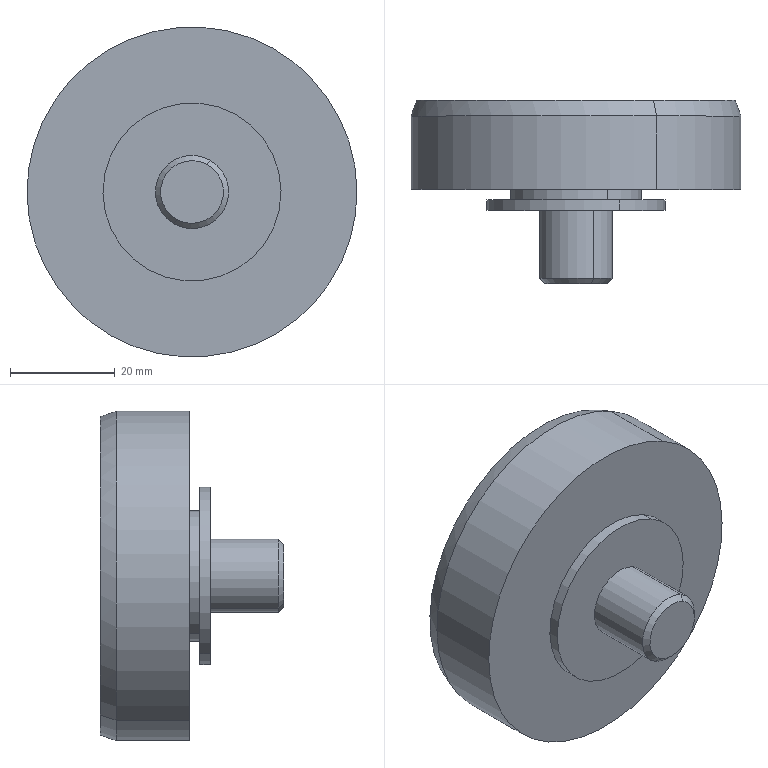Component | SolidWorks | LocatingPinAxis-1 | 1 solid | 17 faces | box 63 x 35 x 63 mm | volume 57605 mm3 | cylinder 8 | plane 5 | cone 4 | commonest cylinder face diameters 14 x2 34 x2 25 x2 63 x2
build123d program:
from build123d import *

# Parameters (mm, degrees)
CHAMFER1_SIZE  = 3
CHAMFER1_SIZE2 = 1.092
CHAMFER2_SIZE  = 1


with BuildPart() as part:
    # Sketch1 → Revolve1 (revolve)
    with BuildSketch(Plane.XY, mode=Mode.PRIVATE) as revolve1_sk:
        Polygon((0, 0), (31.5, 0), (31.5, -17), (12.5, -17), (12.5, -19), (17, -19), (17, -21), (7, -21), (7, -35), (0, -35), align=None)
    revolve(revolve1_sk.sketch.rotate(Axis((0, -35, 0), (0, 1, 0)), 90), axis=Axis((0, -35, 0), (0, 1, 0)))

    # Chamfer1
    chamfer1_edges = [part.edges().sort_by_distance(p)[0] for p in [
        (0, 0, 31.5),
    ]]
    chamfer1_side = [part.faces().sort_by_distance(p)[0] for p in [
        (0, -8.5, 31.5),
    ]]
    chamfer(chamfer1_edges, length=CHAMFER1_SIZE, length2=CHAMFER1_SIZE2, reference=chamfer1_side[0])

    # Chamfer2
    chamfer2_edges = [part.edges().sort_by_distance(p)[0] for p in [
        (0, -35, 7),
    ]]
    chamfer(chamfer2_edges, length=CHAMFER2_SIZE)


solid = part.part

# Placed as in the assembly
solid = solid.moved(Location((0, 226.806, 0), (0, 0, 0)))
STEP:
#1=CARTESIAN_POINT('',(-0.1151,7.551,-0.2063));
#2=VERTEX_POINT('',#1);
#3=CARTESIAN_POINT('',(0.1151,7.551,0.2063));
#4=VERTEX_POINT('',#3);
#5=CARTESIAN_POINT('',(-0.,7.551,0.));
#6=DIRECTION('',(0.,-1.,0.));
#7=DIRECTION('',(-0.4873,0.,-0.8733));
#8=AXIS2_PLACEMENT_3D('',#5,#6,#7);
#9=CIRCLE('',#8,0.2362);
#10=EDGE_CURVE('',#2,#4,#9,.T.);
#11=ORIENTED_EDGE('',*,*,#10,.F.);
#12=CARTESIAN_POINT('',(-0.1343,7.591,-0.2407));
#13=VERTEX_POINT('',#12);
#14=CARTESIAN_POINT('',(-0.1151,7.551,-0.2063));
#15=DIRECTION('',(-0.3445,0.7071,-0.6175));
#16=VECTOR('',#15,39.37);
#17=LINE('',#14,#16);
#18=EDGE_CURVE('',#2,#13,#17,.T.);
#19=ORIENTED_EDGE('',*,*,#18,.T.);
#20=CARTESIAN_POINT('',(0.1343,7.591,0.2407));
#21=VERTEX_POINT('',#20);
#22=CARTESIAN_POINT('',(-0.,7.591,0.));
#23=DIRECTION('',(0.,1.,0.));
#24=DIRECTION('',(-0.4873,0.,-0.8733));
#25=AXIS2_PLACEMENT_3D('',#22,#23,#24);
#26=CIRCLE('',#25,0.2756);
#27=EDGE_CURVE('',#21,#13,#26,.T.);
#28=ORIENTED_EDGE('',*,*,#27,.F.);
#29=CARTESIAN_POINT('',(0.1151,7.551,0.2063));
#30=DIRECTION('',(0.3445,0.7071,0.6175));
#31=VECTOR('',#30,39.37);
#32=LINE('',#29,#31);
#33=EDGE_CURVE('',#4,#21,#32,.T.);
#34=ORIENTED_EDGE('',*,*,#33,.F.);
#35=EDGE_LOOP('',(#11,#19,#28,#34));
#36=FACE_OUTER_BOUND('',#35,.T.);
#37=CARTESIAN_POINT('',(-0.,7.551,0.));
#38=DIRECTION('',(0.,1.,0.));
#39=DIRECTION('',(0.4873,0.,0.8733));
#40=AXIS2_PLACEMENT_3D('',#37,#38,#39);
#41=CONICAL_SURFACE('',#40,0.2362,0.7854);
#42=ADVANCED_FACE('',(#36),#41,.T.);
#43=CARTESIAN_POINT('',(0.5833,8.929,1.045));
#44=VERTEX_POINT('',#43);
#45=CARTESIAN_POINT('',(-0.5833,8.929,-1.045));
#46=VERTEX_POINT('',#45);
#47=CARTESIAN_POINT('',(-0.,8.929,0.));
#48=DIRECTION('',(0.,1.,0.));
#49=DIRECTION('',(0.4873,0.,0.8733));
#50=AXIS2_PLACEMENT_3D('',#47,#48,#49);
#51=CIRCLE('',#50,1.197);
#52=EDGE_CURVE('',#44,#46,#51,.T.);
#53=ORIENTED_EDGE('',*,*,#52,.F.);
#54=CARTESIAN_POINT('',(0.6043,8.811,1.083));
#55=VERTEX_POINT('',#54);
#56=CARTESIAN_POINT('',(0.6043,8.811,1.083));
#57=DIRECTION('',(0.1667,-0.9397,0.2987));
#58=VECTOR('',#57,39.37);
#59=LINE('',#56,#58);
#60=EDGE_CURVE('',#44,#55,#59,.T.);
#61=ORIENTED_EDGE('',*,*,#60,.T.);
#62=CARTESIAN_POINT('',(-0.6043,8.811,-1.083));
#63=VERTEX_POINT('',#62);
#64=CARTESIAN_POINT('',(-0.,8.811,0.));
#65=DIRECTION('',(0.,-1.,0.));
#66=DIRECTION('',(0.4873,0.,0.8733));
#67=AXIS2_PLACEMENT_3D('',#64,#65,#66);
#68=CIRCLE('',#67,1.24);
#69=EDGE_CURVE('',#63,#55,#68,.T.);
#70=ORIENTED_EDGE('',*,*,#69,.F.);
#71=CARTESIAN_POINT('',(-0.6043,8.811,-1.083));
#72=DIRECTION('',(-0.1667,-0.9397,-0.2987));
#73=VECTOR('',#72,39.37);
#74=LINE('',#71,#73);
#75=EDGE_CURVE('',#46,#63,#74,.T.);
#76=ORIENTED_EDGE('',*,*,#75,.F.);
#77=EDGE_LOOP('',(#53,#61,#70,#76));
#78=FACE_OUTER_BOUND('',#77,.T.);
#79=CARTESIAN_POINT('',(-0.,8.811,0.));
#80=DIRECTION('',(0.,-1.,0.));
#81=DIRECTION('',(-0.4873,0.,-0.8733));
#82=AXIS2_PLACEMENT_3D('',#79,#80,#81);
#83=CONICAL_SURFACE('',#82,1.24,0.3491);
#84=ADVANCED_FACE('',(#78),#83,.T.);
#85=CARTESIAN_POINT('',(-0.1343,8.103,-0.2407));
#86=VERTEX_POINT('',#85);
#87=CARTESIAN_POINT('',(0.1343,8.103,0.2407));
#88=VERTEX_POINT('',#87);
#89=CARTESIAN_POINT('',(-0.,8.103,0.));
#90=DIRECTION('',(0.,-1.,0.));
#91=DIRECTION('',(-0.4873,0.,-0.8733));
#92=AXIS2_PLACEMENT_3D('',#89,#90,#91);
#93=CIRCLE('',#92,0.2756);
#94=EDGE_CURVE('',#86,#88,#93,.T.);
#95=ORIENTED_EDGE('',*,*,#94,.T.);
#96=CARTESIAN_POINT('',(0.1343,7.551,0.2407));
#97=DIRECTION('',(0.,-1.,0.));
#98=VECTOR('',#97,39.37);
#99=LINE('',#96,#98);
#100=EDGE_CURVE('',#88,#21,#99,.T.);
#101=ORIENTED_EDGE('',*,*,#100,.T.);
#102=ORIENTED_EDGE('',*,*,#27,.T.);
#103=CARTESIAN_POINT('',(-0.1343,7.551,-0.2407));
#104=DIRECTION('',(0.,-1.,0.));
#105=VECTOR('',#104,39.37);
#106=LINE('',#103,#105);
#107=EDGE_CURVE('',#86,#13,#106,.T.);
#108=ORIENTED_EDGE('',*,*,#107,.F.);
#109=EDGE_LOOP('',(#95,#101,#102,#108));
#110=FACE_OUTER_BOUND('',#109,.T.);
#111=CARTESIAN_POINT('',(-0.,7.551,0.));
#112=DIRECTION('',(0.,-1.,0.));
#113=DIRECTION('',(-0.4873,0.,-0.8733));
#114=AXIS2_PLACEMENT_3D('',#111,#112,#113);
#115=CYLINDRICAL_SURFACE('',#114,0.2756);
#116=ADVANCED_FACE('',(#110),#115,.T.);
#117=CARTESIAN_POINT('',(-0.3261,8.181,-0.5845));
#118=VERTEX_POINT('',#117);
#119=CARTESIAN_POINT('',(0.3261,8.181,0.5845));
#120=VERTEX_POINT('',#119);
#121=CARTESIAN_POINT('',(-0.,8.181,0.));
#122=DIRECTION('',(0.,-1.,0.));
#123=DIRECTION('',(-0.4873,0.,-0.8733));
#124=AXIS2_PLACEMENT_3D('',#121,#122,#123);
#125=CIRCLE('',#124,0.6693);
#126=EDGE_CURVE('',#118,#120,#125,.T.);
#127=ORIENTED_EDGE('',*,*,#126,.T.);
#128=CARTESIAN_POINT('',(0.3261,8.103,0.5845));
#129=VERTEX_POINT('',#128);
#130=CARTESIAN_POINT('',(0.3261,7.551,0.5845));
#131=DIRECTION('',(0.,-1.,0.));
#132=VECTOR('',#131,39.37);
#133=LINE('',#130,#132);
#134=EDGE_CURVE('',#120,#129,#133,.T.);
#135=ORIENTED_EDGE('',*,*,#134,.T.);
#136=CARTESIAN_POINT('',(-0.3261,8.103,-0.5845));
#137=VERTEX_POINT('',#136);
#138=CARTESIAN_POINT('',(-0.,8.103,0.));
#139=DIRECTION('',(0.,-1.,0.));
#140=DIRECTION('',(-0.4873,0.,-0.8733));
#141=AXIS2_PLACEMENT_3D('',#138,#139,#140);
#142=CIRCLE('',#141,0.6693);
#143=EDGE_CURVE('',#137,#129,#142,.T.);
#144=ORIENTED_EDGE('',*,*,#143,.F.);
#145=CARTESIAN_POINT('',(-0.3261,7.551,-0.5845));
#146=DIRECTION('',(0.,-1.,0.));
#147=VECTOR('',#146,39.37);
#148=LINE('',#145,#147);
#149=EDGE_CURVE('',#118,#137,#148,.T.);
#150=ORIENTED_EDGE('',*,*,#149,.F.);
#151=EDGE_LOOP('',(#127,#135,#144,#150));
#152=FACE_OUTER_BOUND('',#151,.T.);
#153=CARTESIAN_POINT('',(-0.,7.551,0.));
#154=DIRECTION('',(0.,-1.,0.));
#155=DIRECTION('',(-0.4873,0.,-0.8733));
#156=AXIS2_PLACEMENT_3D('',#153,#154,#155);
#157=CYLINDRICAL_SURFACE('',#156,0.6693);
#158=ADVANCED_FACE('',(#152),#157,.T.);
#159=CARTESIAN_POINT('',(-0.2398,8.26,-0.4298));
#160=VERTEX_POINT('',#159);
#161=CARTESIAN_POINT('',(0.2398,8.26,0.4298));
#162=VERTEX_POINT('',#161);
#163=CARTESIAN_POINT('',(-0.,8.26,0.));
#164=DIRECTION('',(0.,-1.,0.));
#165=DIRECTION('',(-0.4873,0.,-0.8733));
#166=AXIS2_PLACEMENT_3D('',#163,#164,#165);
#167=CIRCLE('',#166,0.4921);
#168=EDGE_CURVE('',#160,#162,#167,.T.);
#169=ORIENTED_EDGE('',*,*,#168,.T.);
#170=CARTESIAN_POINT('',(0.2398,8.181,0.4298));
#171=VERTEX_POINT('',#170);
#172=CARTESIAN_POINT('',(0.2398,7.551,0.4298));
#173=DIRECTION('',(0.,-1.,0.));
#174=VECTOR('',#173,39.37);
#175=LINE('',#172,#174);
#176=EDGE_CURVE('',#162,#171,#175,.T.);
#177=ORIENTED_EDGE('',*,*,#176,.T.);
#178=CARTESIAN_POINT('',(-0.2398,8.181,-0.4298));
#179=VERTEX_POINT('',#178);
#180=CARTESIAN_POINT('',(-0.,8.181,0.));
#181=DIRECTION('',(0.,-1.,0.));
#182=DIRECTION('',(-0.4873,0.,-0.8733));
#183=AXIS2_PLACEMENT_3D('',#180,#181,#182);
#184=CIRCLE('',#183,0.4921);
#185=EDGE_CURVE('',#179,#171,#184,.T.);
#186=ORIENTED_EDGE('',*,*,#185,.F.);
#187=CARTESIAN_POINT('',(-0.2398,7.551,-0.4298));
#188=DIRECTION('',(0.,-1.,0.));
#189=VECTOR('',#188,39.37);
#190=LINE('',#187,#189);
#191=EDGE_CURVE('',#160,#179,#190,.T.);
#192=ORIENTED_EDGE('',*,*,#191,.F.);
#193=EDGE_LOOP('',(#169,#177,#186,#192));
#194=FACE_OUTER_BOUND('',#193,.T.);
#195=CARTESIAN_POINT('',(-0.,7.551,0.));
#196=DIRECTION('',(0.,-1.,0.));
#197=DIRECTION('',(-0.4873,0.,-0.8733));
#198=AXIS2_PLACEMENT_3D('',#195,#196,#197);
#199=CYLINDRICAL_SURFACE('',#198,0.4921);
#200=ADVANCED_FACE('',(#194),#199,.T.);
#201=ORIENTED_EDGE('',*,*,#69,.T.);
#202=CARTESIAN_POINT('',(0.6043,8.26,1.083));
#203=VERTEX_POINT('',#202);
#204=CARTESIAN_POINT('',(0.6043,7.551,1.083));
#205=DIRECTION('',(0.,-1.,0.));
#206=VECTOR('',#205,39.37);
#207=LINE('',#204,#206);
#208=EDGE_CURVE('',#55,#203,#207,.T.);
#209=ORIENTED_EDGE('',*,*,#208,.T.);
#210=CARTESIAN_POINT('',(-0.6043,8.26,-1.083));
#211=VERTEX_POINT('',#210);
#212=CARTESIAN_POINT('',(-0.,8.26,0.));
#213=DIRECTION('',(0.,-1.,0.));
#214=DIRECTION('',(-0.4873,0.,-0.8733));
#215=AXIS2_PLACEMENT_3D('',#212,#213,#214);
#216=CIRCLE('',#215,1.24);
#217=EDGE_CURVE('',#211,#203,#216,.T.);
#218=ORIENTED_EDGE('',*,*,#217,.F.);
#219=CARTESIAN_POINT('',(-0.6043,7.551,-1.083));
#220=DIRECTION('',(0.,-1.,0.));
#221=VECTOR('',#220,39.37);
#222=LINE('',#219,#221);
#223=EDGE_CURVE('',#63,#211,#222,.T.);
#224=ORIENTED_EDGE('',*,*,#223,.F.);
#225=EDGE_LOOP('',(#201,#209,#218,#224));
#226=FACE_OUTER_BOUND('',#225,.T.);
#227=CARTESIAN_POINT('',(-0.,7.551,0.));
#228=DIRECTION('',(0.,-1.,0.));
#229=DIRECTION('',(-0.4873,0.,-0.8733));
#230=AXIS2_PLACEMENT_3D('',#227,#228,#229);
#231=CYLINDRICAL_SURFACE('',#230,1.24);
#232=ADVANCED_FACE('',(#226),#231,.T.);
#233=CARTESIAN_POINT('',(-0.,8.929,0.));
#234=DIRECTION('',(0.,1.,0.));
#235=DIRECTION('',(0.4873,0.,0.8733));
#236=AXIS2_PLACEMENT_3D('',#233,#234,#235);
#237=CIRCLE('',#236,1.197);
#238=EDGE_CURVE('',#46,#44,#237,.T.);
#239=ORIENTED_EDGE('',*,*,#238,.T.);
#240=ORIENTED_EDGE('',*,*,#52,.T.);
#241=EDGE_LOOP('',(#239,#240));
#242=FACE_OUTER_BOUND('',#241,.T.);
#243=CARTESIAN_POINT('',(-0.,8.929,0.));
#244=DIRECTION('',(0.,1.,0.));
#245=DIRECTION('',(0.4873,0.,0.8733));
#246=AXIS2_PLACEMENT_3D('',#243,#244,#245);
#247=PLANE('',#246);
#248=ADVANCED_FACE('',(#242),#247,.T.);
#249=ORIENTED_EDGE('',*,*,#208,.F.);
#250=CARTESIAN_POINT('',(-0.,8.811,0.));
#251=DIRECTION('',(0.,-1.,0.));
#252=DIRECTION('',(0.4873,0.,0.8733));
#253=AXIS2_PLACEMENT_3D('',#250,#251,#252);
#254=CIRCLE('',#253,1.24);
#255=EDGE_CURVE('',#55,#63,#254,.T.);
#256=ORIENTED_EDGE('',*,*,#255,.T.);
#257=ORIENTED_EDGE('',*,*,#223,.T.);
#258=CARTESIAN_POINT('',(-0.,8.26,0.));
#259=DIRECTION('',(0.,-1.,0.));
#260=DIRECTION('',(-0.4873,0.,-0.8733));
#261=AXIS2_PLACEMENT_3D('',#258,#259,#260);
#262=CIRCLE('',#261,1.24);
#263=EDGE_CURVE('',#203,#211,#262,.T.);
#264=ORIENTED_EDGE('',*,*,#263,.F.);
#265=EDGE_LOOP('',(#249,#256,#257,#264));
#266=FACE_OUTER_BOUND('',#265,.T.);
#267=CARTESIAN_POINT('',(-0.,7.551,0.));
#268=DIRECTION('',(0.,-1.,0.));
#269=DIRECTION('',(-0.4873,0.,-0.8733));
#270=AXIS2_PLACEMENT_3D('',#267,#268,#269);
#271=CYLINDRICAL_SURFACE('',#270,1.24);
#272=ADVANCED_FACE('',(#266),#271,.T.);
#273=ORIENTED_EDGE('',*,*,#217,.T.);
#274=ORIENTED_EDGE('',*,*,#263,.T.);
#275=EDGE_LOOP('',(#273,#274));
#276=FACE_OUTER_BOUND('',#275,.T.);
#277=ORIENTED_EDGE('',*,*,#168,.F.);
#278=CARTESIAN_POINT('',(-0.,8.26,0.));
#279=DIRECTION('',(0.,-1.,0.));
#280=DIRECTION('',(-0.4873,0.,-0.8733));
#281=AXIS2_PLACEMENT_3D('',#278,#279,#280);
#282=CIRCLE('',#281,0.4921);
#283=EDGE_CURVE('',#162,#160,#282,.T.);
#284=ORIENTED_EDGE('',*,*,#283,.F.);
#285=EDGE_LOOP('',(#277,#284));
#286=FACE_BOUND('',#285,.T.);
#287=CARTESIAN_POINT('',(0.4298,8.26,-0.2398));
#288=DIRECTION('',(0.,-1.,0.));
#289=DIRECTION('',(-0.4873,0.,-0.8733));
#290=AXIS2_PLACEMENT_3D('',#287,#288,#289);
#291=PLANE('',#290);
#292=ADVANCED_FACE('',(#276,#286),#291,.T.);
#293=ORIENTED_EDGE('',*,*,#176,.F.);
#294=ORIENTED_EDGE('',*,*,#283,.T.);
#295=ORIENTED_EDGE('',*,*,#191,.T.);
#296=CARTESIAN_POINT('',(-0.,8.181,0.));
#297=DIRECTION('',(0.,-1.,0.));
#298=DIRECTION('',(-0.4873,0.,-0.8733));
#299=AXIS2_PLACEMENT_3D('',#296,#297,#298);
#300=CIRCLE('',#299,0.4921);
#301=EDGE_CURVE('',#171,#179,#300,.T.);
#302=ORIENTED_EDGE('',*,*,#301,.F.);
#303=EDGE_LOOP('',(#293,#294,#295,#302));
#304=FACE_OUTER_BOUND('',#303,.T.);
#305=CARTESIAN_POINT('',(-0.,7.551,0.));
#306=DIRECTION('',(0.,-1.,0.));
#307=DIRECTION('',(-0.4873,0.,-0.8733));
#308=AXIS2_PLACEMENT_3D('',#305,#306,#307);
#309=CYLINDRICAL_SURFACE('',#308,0.4921);
#310=ADVANCED_FACE('',(#304),#309,.T.);
#311=ORIENTED_EDGE('',*,*,#185,.T.);
#312=ORIENTED_EDGE('',*,*,#301,.T.);
#313=EDGE_LOOP('',(#311,#312));
#314=FACE_BOUND('',#313,.T.);
#315=ORIENTED_EDGE('',*,*,#126,.F.);
#316=CARTESIAN_POINT('',(-0.,8.181,0.));
#317=DIRECTION('',(0.,-1.,0.));
#318=DIRECTION('',(-0.4873,0.,-0.8733));
#319=AXIS2_PLACEMENT_3D('',#316,#317,#318);
#320=CIRCLE('',#319,0.6693);
#321=EDGE_CURVE('',#120,#118,#320,.T.);
#322=ORIENTED_EDGE('',*,*,#321,.F.);
#323=EDGE_LOOP('',(#315,#322));
#324=FACE_OUTER_BOUND('',#323,.T.);
#325=CARTESIAN_POINT('',(0.4298,8.181,-0.2398));
#326=DIRECTION('',(0.,1.,0.));
#327=DIRECTION('',(0.4873,0.,0.8733));
#328=AXIS2_PLACEMENT_3D('',#325,#326,#327);
#329=PLANE('',#328);
#330=ADVANCED_FACE('',(#314,#324),#329,.T.);
#331=ORIENTED_EDGE('',*,*,#134,.F.);
#332=ORIENTED_EDGE('',*,*,#321,.T.);
#333=ORIENTED_EDGE('',*,*,#149,.T.);
#334=CARTESIAN_POINT('',(-0.,8.103,0.));
#335=DIRECTION('',(0.,-1.,0.));
#336=DIRECTION('',(-0.4873,0.,-0.8733));
#337=AXIS2_PLACEMENT_3D('',#334,#335,#336);
#338=CIRCLE('',#337,0.6693);
#339=EDGE_CURVE('',#129,#137,#338,.T.);
#340=ORIENTED_EDGE('',*,*,#339,.F.);
#341=EDGE_LOOP('',(#331,#332,#333,#340));
#342=FACE_OUTER_BOUND('',#341,.T.);
#343=CARTESIAN_POINT('',(-0.,7.551,0.));
#344=DIRECTION('',(0.,-1.,0.));
#345=DIRECTION('',(-0.4873,0.,-0.8733));
#346=AXIS2_PLACEMENT_3D('',#343,#344,#345);
#347=CYLINDRICAL_SURFACE('',#346,0.6693);
#348=ADVANCED_FACE('',(#342),#347,.T.);
#349=ORIENTED_EDGE('',*,*,#143,.T.);
#350=ORIENTED_EDGE('',*,*,#339,.T.);
#351=EDGE_LOOP('',(#349,#350));
#352=FACE_OUTER_BOUND('',#351,.T.);
#353=ORIENTED_EDGE('',*,*,#94,.F.);
#354=CARTESIAN_POINT('',(-0.,8.103,0.));
#355=DIRECTION('',(0.,-1.,0.));
#356=DIRECTION('',(-0.4873,0.,-0.8733));
#357=AXIS2_PLACEMENT_3D('',#354,#355,#356);
#358=CIRCLE('',#357,0.2756);
#359=EDGE_CURVE('',#88,#86,#358,.T.);
#360=ORIENTED_EDGE('',*,*,#359,.F.);
#361=EDGE_LOOP('',(#353,#360));
#362=FACE_BOUND('',#361,.T.);
#363=CARTESIAN_POINT('',(0.5845,8.103,-0.3261));
#364=DIRECTION('',(0.,-1.,0.));
#365=DIRECTION('',(-0.4873,0.,-0.8733));
#366=AXIS2_PLACEMENT_3D('',#363,#364,#365);
#367=PLANE('',#366);
#368=ADVANCED_FACE('',(#352,#362),#367,.T.);
#369=ORIENTED_EDGE('',*,*,#100,.F.);
#370=ORIENTED_EDGE('',*,*,#359,.T.);
#371=ORIENTED_EDGE('',*,*,#107,.T.);
#372=CARTESIAN_POINT('',(-0.,7.591,0.));
#373=DIRECTION('',(0.,1.,0.));
#374=DIRECTION('',(-0.4873,0.,-0.8733));
#375=AXIS2_PLACEMENT_3D('',#372,#373,#374);
#376=CIRCLE('',#375,0.2756);
#377=EDGE_CURVE('',#13,#21,#376,.T.);
#378=ORIENTED_EDGE('',*,*,#377,.T.);
#379=EDGE_LOOP('',(#369,#370,#371,#378));
#380=FACE_OUTER_BOUND('',#379,.T.);
#381=CARTESIAN_POINT('',(-0.,7.551,0.));
#382=DIRECTION('',(0.,-1.,0.));
#383=DIRECTION('',(-0.4873,0.,-0.8733));
#384=AXIS2_PLACEMENT_3D('',#381,#382,#383);
#385=CYLINDRICAL_SURFACE('',#384,0.2756);
#386=ADVANCED_FACE('',(#380),#385,.T.);
#387=CARTESIAN_POINT('',(-0.,7.551,0.));
#388=DIRECTION('',(0.,-1.,0.));
#389=DIRECTION('',(-0.4873,0.,-0.8733));
#390=AXIS2_PLACEMENT_3D('',#387,#388,#389);
#391=CIRCLE('',#390,0.2362);
#392=EDGE_CURVE('',#4,#2,#391,.T.);
#393=ORIENTED_EDGE('',*,*,#392,.T.);
#394=ORIENTED_EDGE('',*,*,#10,.T.);
#395=EDGE_LOOP('',(#393,#394));
#396=FACE_OUTER_BOUND('',#395,.T.);
#397=CARTESIAN_POINT('',(0.2407,7.551,-0.1343));
#398=DIRECTION('',(0.,-1.,0.));
#399=DIRECTION('',(-0.4873,0.,-0.8733));
#400=AXIS2_PLACEMENT_3D('',#397,#398,#399);
#401=PLANE('',#400);
#402=ADVANCED_FACE('',(#396),#401,.T.);
#403=ORIENTED_EDGE('',*,*,#60,.F.);
#404=ORIENTED_EDGE('',*,*,#238,.F.);
#405=ORIENTED_EDGE('',*,*,#75,.T.);
#406=ORIENTED_EDGE('',*,*,#255,.F.);
#407=EDGE_LOOP('',(#403,#404,#405,#406));
#408=FACE_OUTER_BOUND('',#407,.T.);
#409=CARTESIAN_POINT('',(-0.,8.811,0.));
#410=DIRECTION('',(0.,-1.,0.));
#411=DIRECTION('',(-0.4873,0.,-0.8733));
#412=AXIS2_PLACEMENT_3D('',#409,#410,#411);
#413=CONICAL_SURFACE('',#412,1.24,0.3491);
#414=ADVANCED_FACE('',(#408),#413,.T.);
#415=ORIENTED_EDGE('',*,*,#18,.F.);
#416=ORIENTED_EDGE('',*,*,#392,.F.);
#417=ORIENTED_EDGE('',*,*,#33,.T.);
#418=ORIENTED_EDGE('',*,*,#377,.F.);
#419=EDGE_LOOP('',(#415,#416,#417,#418));
#420=FACE_OUTER_BOUND('',#419,.T.);
#421=CARTESIAN_POINT('',(-0.,7.551,0.));
#422=DIRECTION('',(0.,1.,0.));
#423=DIRECTION('',(0.4873,0.,0.8733));
#424=AXIS2_PLACEMENT_3D('',#421,#422,#423);
#425=CONICAL_SURFACE('',#424,0.2362,0.7854);
#426=ADVANCED_FACE('',(#420),#425,.T.);
#427=CLOSED_SHELL('',(#42,#84,#116,#158,#200,#232,#248,#272,#292,#310,#330,#348,#368,#386,#402,#414,#426));
#428=MANIFOLD_SOLID_BREP('',#427);
#429=CARTESIAN_POINT('',(0.,0.,0.));
#430=DIRECTION('',(0.,0.,1.));
#431=DIRECTION('',(1.,0.,0.));
#432=AXIS2_PLACEMENT_3D('',#429,#430,#431);
#433=(LENGTH_UNIT()NAMED_UNIT(*)SI_UNIT($,.METRE.));
#434=LENGTH_MEASURE_WITH_UNIT(LENGTH_MEASURE(0.0254),#433);
#435=DIMENSIONAL_EXPONENTS(1.,0.,0.,0.,0.,0.,0.);
#436=(CONVERSION_BASED_UNIT('',#434)LENGTH_UNIT()NAMED_UNIT(#435));
#437=UNCERTAINTY_MEASURE_WITH_UNIT(LENGTH_MEASURE(0.00001),#436,'','');
#438=(NAMED_UNIT(*)PLANE_ANGLE_UNIT()SI_UNIT($,.RADIAN.));
#439=(NAMED_UNIT(*)SI_UNIT($,.STERADIAN.)SOLID_ANGLE_UNIT());
#440=(GEOMETRIC_REPRESENTATION_CONTEXT(3)GLOBAL_UNCERTAINTY_ASSIGNED_CONTEXT((#437))GLOBAL_UNIT_ASSIGNED_CONTEXT((#436,#438,#439))REPRESENTATION_CONTEXT('',''));
#441=ADVANCED_BREP_SHAPE_REPRESENTATION('',(#428,#432),#440);
#442=COLOUR_RGB('',0.7922,0.8196,0.9333);
#443=FILL_AREA_STYLE_COLOUR('',#442);
#444=FILL_AREA_STYLE('',(#443));
#445=SURFACE_STYLE_FILL_AREA(#444);
#446=SURFACE_SIDE_STYLE('',(#445));
#447=SURFACE_STYLE_USAGE(.BOTH.,#446);
#448=PRESENTATION_STYLE_ASSIGNMENT((#447));
#449=STYLED_ITEM('',(#448),#428);
#450=(LENGTH_UNIT()NAMED_UNIT(*)SI_UNIT($,.METRE.));
#451=LENGTH_MEASURE_WITH_UNIT(LENGTH_MEASURE(0.0254),#450);
#452=DIMENSIONAL_EXPONENTS(1.,0.,0.,0.,0.,0.,0.);
#453=(CONVERSION_BASED_UNIT('',#451)LENGTH_UNIT()NAMED_UNIT(#452));
#454=UNCERTAINTY_MEASURE_WITH_UNIT(LENGTH_MEASURE(0.00001),#453,'','');
#455=(NAMED_UNIT(*)PLANE_ANGLE_UNIT()SI_UNIT($,.RADIAN.));
#456=(NAMED_UNIT(*)SI_UNIT($,.STERADIAN.)SOLID_ANGLE_UNIT());
#457=(GEOMETRIC_REPRESENTATION_CONTEXT(3)GLOBAL_UNCERTAINTY_ASSIGNED_CONTEXT((#454))GLOBAL_UNIT_ASSIGNED_CONTEXT((#453,#455,#456))REPRESENTATION_CONTEXT('',''));
#458=MECHANICAL_DESIGN_GEOMETRIC_PRESENTATION_REPRESENTATION('',(#449),#457);
#459=PRESENTATION_LAYER_ASSIGNMENT('','',(#449));